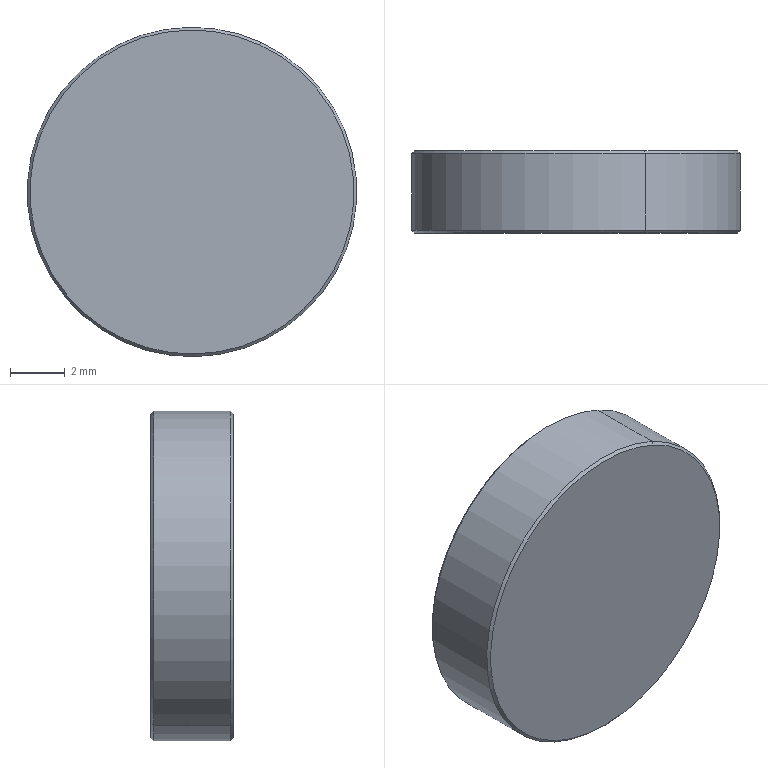Component | SolidWorks | GbgbMagnetF8-1 | 1 solid | 8 faces | box 12 x 3 x 12 mm | volume 339 mm3 | cone 4 | cylinder 2 | plane 2 | commonest cylinder face diameters 12 x2
build123d program:
from build123d import *

# Parameters (mm, degrees)
SKETCH1_R           = 6
BOSS_EXTRUDE1_DEPTH = 1.5
CHAMFER1_SIZE       = 0.1


with BuildPart() as part:
    # Sketch1 → Boss-Extrude1 (new, symmetric)
    with BuildSketch(Plane(origin=(0, 0, 0), x_dir=(1, 0, 0), z_dir=(0, 1, 0))):
        with Locations(Location((0, 0, 0), (0, 0, 270))):
            Circle(SKETCH1_R)
    extrude(amount=BOSS_EXTRUDE1_DEPTH, both=True)

    # Chamfer1
    chamfer1_edges = [part.edges().sort_by_distance(p)[0] for p in [
        (0, -1.5, -6),
        (0, 1.5, -6),
    ]]
    chamfer(chamfer1_edges, length=CHAMFER1_SIZE)


solid = part.part

# Placed as in the assembly
solid = solid.moved(Location((80.446, 385.84, 408.232), (0, 0, 0)))
STEP:
#1=COLOUR_RGB('',0.7922,0.8196,0.9333);
#2=FILL_AREA_STYLE_COLOUR('',#1);
#3=FILL_AREA_STYLE('',(#2));
#4=SURFACE_STYLE_FILL_AREA(#3);
#5=SURFACE_SIDE_STYLE('',(#4));
#6=SURFACE_STYLE_USAGE(.BOTH.,#5);
#7=PRESENTATION_STYLE_ASSIGNMENT((#6));
#8=CARTESIAN_POINT('',(3.07,15.132,15.861));
#9=VERTEX_POINT('',#8);
#10=CARTESIAN_POINT('',(3.265,15.132,16.283));
#11=VERTEX_POINT('',#10);
#12=CARTESIAN_POINT('',(3.167,15.132,16.072));
#13=DIRECTION('',(-0.,-1.,0.));
#14=DIRECTION('',(-0.4196,0.,-0.9077));
#15=AXIS2_PLACEMENT_3D('',#12,#13,#14);
#16=CIRCLE('',#15,0.2323);
#17=EDGE_CURVE('',#9,#11,#16,.T.);
#18=ORIENTED_EDGE('',*,*,#17,.F.);
#19=CARTESIAN_POINT('',(3.068,15.135,15.858));
#20=VERTEX_POINT('',#19);
#21=CARTESIAN_POINT('',(3.07,15.132,15.861));
#22=DIRECTION('',(-0.2967,0.7071,-0.6418));
#23=VECTOR('',#22,39.37);
#24=LINE('',#21,#23);
#25=EDGE_CURVE('',#9,#20,#24,.T.);
#26=ORIENTED_EDGE('',*,*,#25,.T.);
#27=CARTESIAN_POINT('',(3.266,15.135,16.287));
#28=VERTEX_POINT('',#27);
#29=CARTESIAN_POINT('',(3.167,15.135,16.072));
#30=DIRECTION('',(0.,1.,-0.));
#31=DIRECTION('',(-0.4196,0.,-0.9077));
#32=AXIS2_PLACEMENT_3D('',#29,#30,#31);
#33=CIRCLE('',#32,0.2362);
#34=EDGE_CURVE('',#28,#20,#33,.T.);
#35=ORIENTED_EDGE('',*,*,#34,.F.);
#36=CARTESIAN_POINT('',(3.265,15.132,16.283));
#37=DIRECTION('',(0.2967,0.7071,0.6418));
#38=VECTOR('',#37,39.37);
#39=LINE('',#36,#38);
#40=EDGE_CURVE('',#11,#28,#39,.T.);
#41=ORIENTED_EDGE('',*,*,#40,.F.);
#42=EDGE_LOOP('',(#18,#26,#35,#41));
#43=FACE_OUTER_BOUND('',#42,.T.);
#44=CARTESIAN_POINT('',(3.167,15.132,16.072));
#45=DIRECTION('',(0.,1.,-0.));
#46=DIRECTION('',(0.4196,0.,0.9077));
#47=AXIS2_PLACEMENT_3D('',#44,#45,#46);
#48=CONICAL_SURFACE('',#47,0.2323,0.7854);
#49=ADVANCED_FACE('',(#43),#48,.T.);
#50=CARTESIAN_POINT('',(3.265,15.25,16.283));
#51=VERTEX_POINT('',#50);
#52=CARTESIAN_POINT('',(3.07,15.25,15.861));
#53=VERTEX_POINT('',#52);
#54=CARTESIAN_POINT('',(3.167,15.25,16.072));
#55=DIRECTION('',(0.,1.,-0.));
#56=DIRECTION('',(-0.4196,0.,-0.9077));
#57=AXIS2_PLACEMENT_3D('',#54,#55,#56);
#58=CIRCLE('',#57,0.2323);
#59=EDGE_CURVE('',#51,#53,#58,.T.);
#60=ORIENTED_EDGE('',*,*,#59,.F.);
#61=CARTESIAN_POINT('',(3.266,15.246,16.287));
#62=VERTEX_POINT('',#61);
#63=CARTESIAN_POINT('',(3.266,15.246,16.287));
#64=DIRECTION('',(0.2967,-0.7071,0.6418));
#65=VECTOR('',#64,39.37);
#66=LINE('',#63,#65);
#67=EDGE_CURVE('',#51,#62,#66,.T.);
#68=ORIENTED_EDGE('',*,*,#67,.T.);
#69=CARTESIAN_POINT('',(3.068,15.246,15.858));
#70=VERTEX_POINT('',#69);
#71=CARTESIAN_POINT('',(3.167,15.246,16.072));
#72=DIRECTION('',(-0.,-1.,0.));
#73=DIRECTION('',(-0.4196,0.,-0.9077));
#74=AXIS2_PLACEMENT_3D('',#71,#72,#73);
#75=CIRCLE('',#74,0.2362);
#76=EDGE_CURVE('',#70,#62,#75,.T.);
#77=ORIENTED_EDGE('',*,*,#76,.F.);
#78=CARTESIAN_POINT('',(3.068,15.246,15.858));
#79=DIRECTION('',(-0.2967,-0.7071,-0.6418));
#80=VECTOR('',#79,39.37);
#81=LINE('',#78,#80);
#82=EDGE_CURVE('',#53,#70,#81,.T.);
#83=ORIENTED_EDGE('',*,*,#82,.F.);
#84=EDGE_LOOP('',(#60,#68,#77,#83));
#85=FACE_OUTER_BOUND('',#84,.T.);
#86=CARTESIAN_POINT('',(3.167,15.246,16.072));
#87=DIRECTION('',(-0.,-1.,0.));
#88=DIRECTION('',(-0.4196,0.,-0.9077));
#89=AXIS2_PLACEMENT_3D('',#86,#87,#88);
#90=CONICAL_SURFACE('',#89,0.2362,0.7854);
#91=ADVANCED_FACE('',(#85),#90,.T.);
#92=ORIENTED_EDGE('',*,*,#34,.T.);
#93=CARTESIAN_POINT('',(3.068,15.132,15.858));
#94=DIRECTION('',(0.,1.,-0.));
#95=VECTOR('',#94,39.37);
#96=LINE('',#93,#95);
#97=EDGE_CURVE('',#20,#70,#96,.T.);
#98=ORIENTED_EDGE('',*,*,#97,.T.);
#99=ORIENTED_EDGE('',*,*,#76,.T.);
#100=CARTESIAN_POINT('',(3.266,15.132,16.287));
#101=DIRECTION('',(0.,1.,-0.));
#102=VECTOR('',#101,39.37);
#103=LINE('',#100,#102);
#104=EDGE_CURVE('',#28,#62,#103,.T.);
#105=ORIENTED_EDGE('',*,*,#104,.F.);
#106=EDGE_LOOP('',(#92,#98,#99,#105));
#107=FACE_OUTER_BOUND('',#106,.T.);
#108=CARTESIAN_POINT('',(3.167,15.132,16.072));
#109=DIRECTION('',(0.,1.,-0.));
#110=DIRECTION('',(0.4196,0.,0.9077));
#111=AXIS2_PLACEMENT_3D('',#108,#109,#110);
#112=CYLINDRICAL_SURFACE('',#111,0.2362);
#113=ADVANCED_FACE('',(#107),#112,.T.);
#114=ORIENTED_EDGE('',*,*,#97,.F.);
#115=CARTESIAN_POINT('',(3.167,15.135,16.072));
#116=DIRECTION('',(0.,1.,-0.));
#117=DIRECTION('',(-0.4196,0.,-0.9077));
#118=AXIS2_PLACEMENT_3D('',#115,#116,#117);
#119=CIRCLE('',#118,0.2362);
#120=EDGE_CURVE('',#20,#28,#119,.T.);
#121=ORIENTED_EDGE('',*,*,#120,.T.);
#122=ORIENTED_EDGE('',*,*,#104,.T.);
#123=CARTESIAN_POINT('',(3.167,15.246,16.072));
#124=DIRECTION('',(-0.,-1.,0.));
#125=DIRECTION('',(-0.4196,0.,-0.9077));
#126=AXIS2_PLACEMENT_3D('',#123,#124,#125);
#127=CIRCLE('',#126,0.2362);
#128=EDGE_CURVE('',#62,#70,#127,.T.);
#129=ORIENTED_EDGE('',*,*,#128,.T.);
#130=EDGE_LOOP('',(#114,#121,#122,#129));
#131=FACE_OUTER_BOUND('',#130,.T.);
#132=CARTESIAN_POINT('',(3.167,15.132,16.072));
#133=DIRECTION('',(0.,1.,-0.));
#134=DIRECTION('',(0.4196,0.,0.9077));
#135=AXIS2_PLACEMENT_3D('',#132,#133,#134);
#136=CYLINDRICAL_SURFACE('',#135,0.2362);
#137=ADVANCED_FACE('',(#131),#136,.T.);
#138=CARTESIAN_POINT('',(3.167,15.132,16.072));
#139=DIRECTION('',(-0.,-1.,0.));
#140=DIRECTION('',(-0.4196,0.,-0.9077));
#141=AXIS2_PLACEMENT_3D('',#138,#139,#140);
#142=CIRCLE('',#141,0.2323);
#143=EDGE_CURVE('',#11,#9,#142,.T.);
#144=ORIENTED_EDGE('',*,*,#143,.T.);
#145=ORIENTED_EDGE('',*,*,#17,.T.);
#146=EDGE_LOOP('',(#144,#145));
#147=FACE_OUTER_BOUND('',#146,.T.);
#148=CARTESIAN_POINT('',(3.167,15.132,16.072));
#149=DIRECTION('',(-0.,-1.,0.));
#150=DIRECTION('',(-0.4196,0.,-0.9077));
#151=AXIS2_PLACEMENT_3D('',#148,#149,#150);
#152=PLANE('',#151);
#153=ADVANCED_FACE('',(#147),#152,.T.);
#154=CARTESIAN_POINT('',(3.167,15.25,16.072));
#155=DIRECTION('',(0.,1.,-0.));
#156=DIRECTION('',(-0.4196,0.,-0.9077));
#157=AXIS2_PLACEMENT_3D('',#154,#155,#156);
#158=CIRCLE('',#157,0.2323);
#159=EDGE_CURVE('',#53,#51,#158,.T.);
#160=ORIENTED_EDGE('',*,*,#159,.T.);
#161=ORIENTED_EDGE('',*,*,#59,.T.);
#162=EDGE_LOOP('',(#160,#161));
#163=FACE_OUTER_BOUND('',#162,.T.);
#164=CARTESIAN_POINT('',(3.167,15.25,16.072));
#165=DIRECTION('',(-0.,-1.,0.));
#166=DIRECTION('',(-0.4196,0.,-0.9077));
#167=AXIS2_PLACEMENT_3D('',#164,#165,#166);
#168=PLANE('',#167);
#169=ADVANCED_FACE('',(#163),#168,.F.);
#170=ORIENTED_EDGE('',*,*,#67,.F.);
#171=ORIENTED_EDGE('',*,*,#159,.F.);
#172=ORIENTED_EDGE('',*,*,#82,.T.);
#173=ORIENTED_EDGE('',*,*,#128,.F.);
#174=EDGE_LOOP('',(#170,#171,#172,#173));
#175=FACE_OUTER_BOUND('',#174,.T.);
#176=CARTESIAN_POINT('',(3.167,15.246,16.072));
#177=DIRECTION('',(-0.,-1.,0.));
#178=DIRECTION('',(-0.4196,0.,-0.9077));
#179=AXIS2_PLACEMENT_3D('',#176,#177,#178);
#180=CONICAL_SURFACE('',#179,0.2362,0.7854);
#181=ADVANCED_FACE('',(#175),#180,.T.);
#182=ORIENTED_EDGE('',*,*,#25,.F.);
#183=ORIENTED_EDGE('',*,*,#143,.F.);
#184=ORIENTED_EDGE('',*,*,#40,.T.);
#185=ORIENTED_EDGE('',*,*,#120,.F.);
#186=EDGE_LOOP('',(#182,#183,#184,#185));
#187=FACE_OUTER_BOUND('',#186,.T.);
#188=CARTESIAN_POINT('',(3.167,15.132,16.072));
#189=DIRECTION('',(0.,1.,-0.));
#190=DIRECTION('',(0.4196,0.,0.9077));
#191=AXIS2_PLACEMENT_3D('',#188,#189,#190);
#192=CONICAL_SURFACE('',#191,0.2323,0.7854);
#193=ADVANCED_FACE('',(#187),#192,.T.);
#194=CLOSED_SHELL('',(#49,#91,#113,#137,#153,#169,#181,#193));
#195=MANIFOLD_SOLID_BREP('',#194);
#196=STYLED_ITEM('',(#7),#195);
#197=PRESENTATION_LAYER_ASSIGNMENT('','',(#196));
#198=CARTESIAN_POINT('',(0.,0.,0.));
#199=DIRECTION('',(0.,0.,1.));
#200=DIRECTION('',(1.,0.,0.));
#201=AXIS2_PLACEMENT_3D('',#198,#199,#200);
#202=(LENGTH_UNIT()NAMED_UNIT(*)SI_UNIT($,.METRE.));
#203=LENGTH_MEASURE_WITH_UNIT(LENGTH_MEASURE(0.0254),#202);
#204=DIMENSIONAL_EXPONENTS(1.,0.,0.,0.,0.,0.,0.);
#205=(CONVERSION_BASED_UNIT('',#203)LENGTH_UNIT()NAMED_UNIT(#204));
#206=UNCERTAINTY_MEASURE_WITH_UNIT(LENGTH_MEASURE(0.00001),#205,'','');
#207=(NAMED_UNIT(*)PLANE_ANGLE_UNIT()SI_UNIT($,.RADIAN.));
#208=(NAMED_UNIT(*)SI_UNIT($,.STERADIAN.)SOLID_ANGLE_UNIT());
#209=(GEOMETRIC_REPRESENTATION_CONTEXT(3)GLOBAL_UNCERTAINTY_ASSIGNED_CONTEXT((#206))GLOBAL_UNIT_ASSIGNED_CONTEXT((#205,#207,#208))REPRESENTATION_CONTEXT('',''));
#210=ADVANCED_BREP_SHAPE_REPRESENTATION('',(#195,#201),#209);
#211=(LENGTH_UNIT()NAMED_UNIT(*)SI_UNIT($,.METRE.));
#212=LENGTH_MEASURE_WITH_UNIT(LENGTH_MEASURE(0.0254),#211);
#213=DIMENSIONAL_EXPONENTS(1.,0.,0.,0.,0.,0.,0.);
#214=(CONVERSION_BASED_UNIT('',#212)LENGTH_UNIT()NAMED_UNIT(#213));
#215=UNCERTAINTY_MEASURE_WITH_UNIT(LENGTH_MEASURE(0.00001),#214,'','');
#216=(NAMED_UNIT(*)PLANE_ANGLE_UNIT()SI_UNIT($,.RADIAN.));
#217=(NAMED_UNIT(*)SI_UNIT($,.STERADIAN.)SOLID_ANGLE_UNIT());
#218=(GEOMETRIC_REPRESENTATION_CONTEXT(3)GLOBAL_UNCERTAINTY_ASSIGNED_CONTEXT((#215))GLOBAL_UNIT_ASSIGNED_CONTEXT((#214,#216,#217))REPRESENTATION_CONTEXT('',''));
#219=MECHANICAL_DESIGN_GEOMETRIC_PRESENTATION_REPRESENTATION('',(#196),#218);